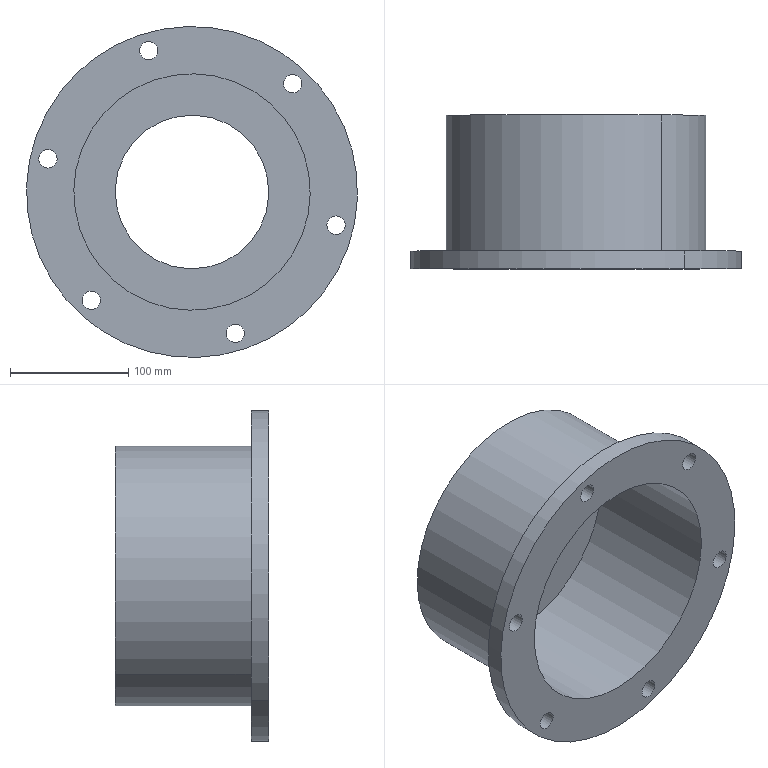Component | SolidWorks | BearingOuterMountingSleeve-1 | 1 solid | 42 faces | box 280 x 130 x 280 mm | volume 1373946 mm3 | cylinder 32 | plane 10 | commonest cylinder face diameters 24 x12 15.5 x12 130 x2 220 x2 200 x2 280 x2